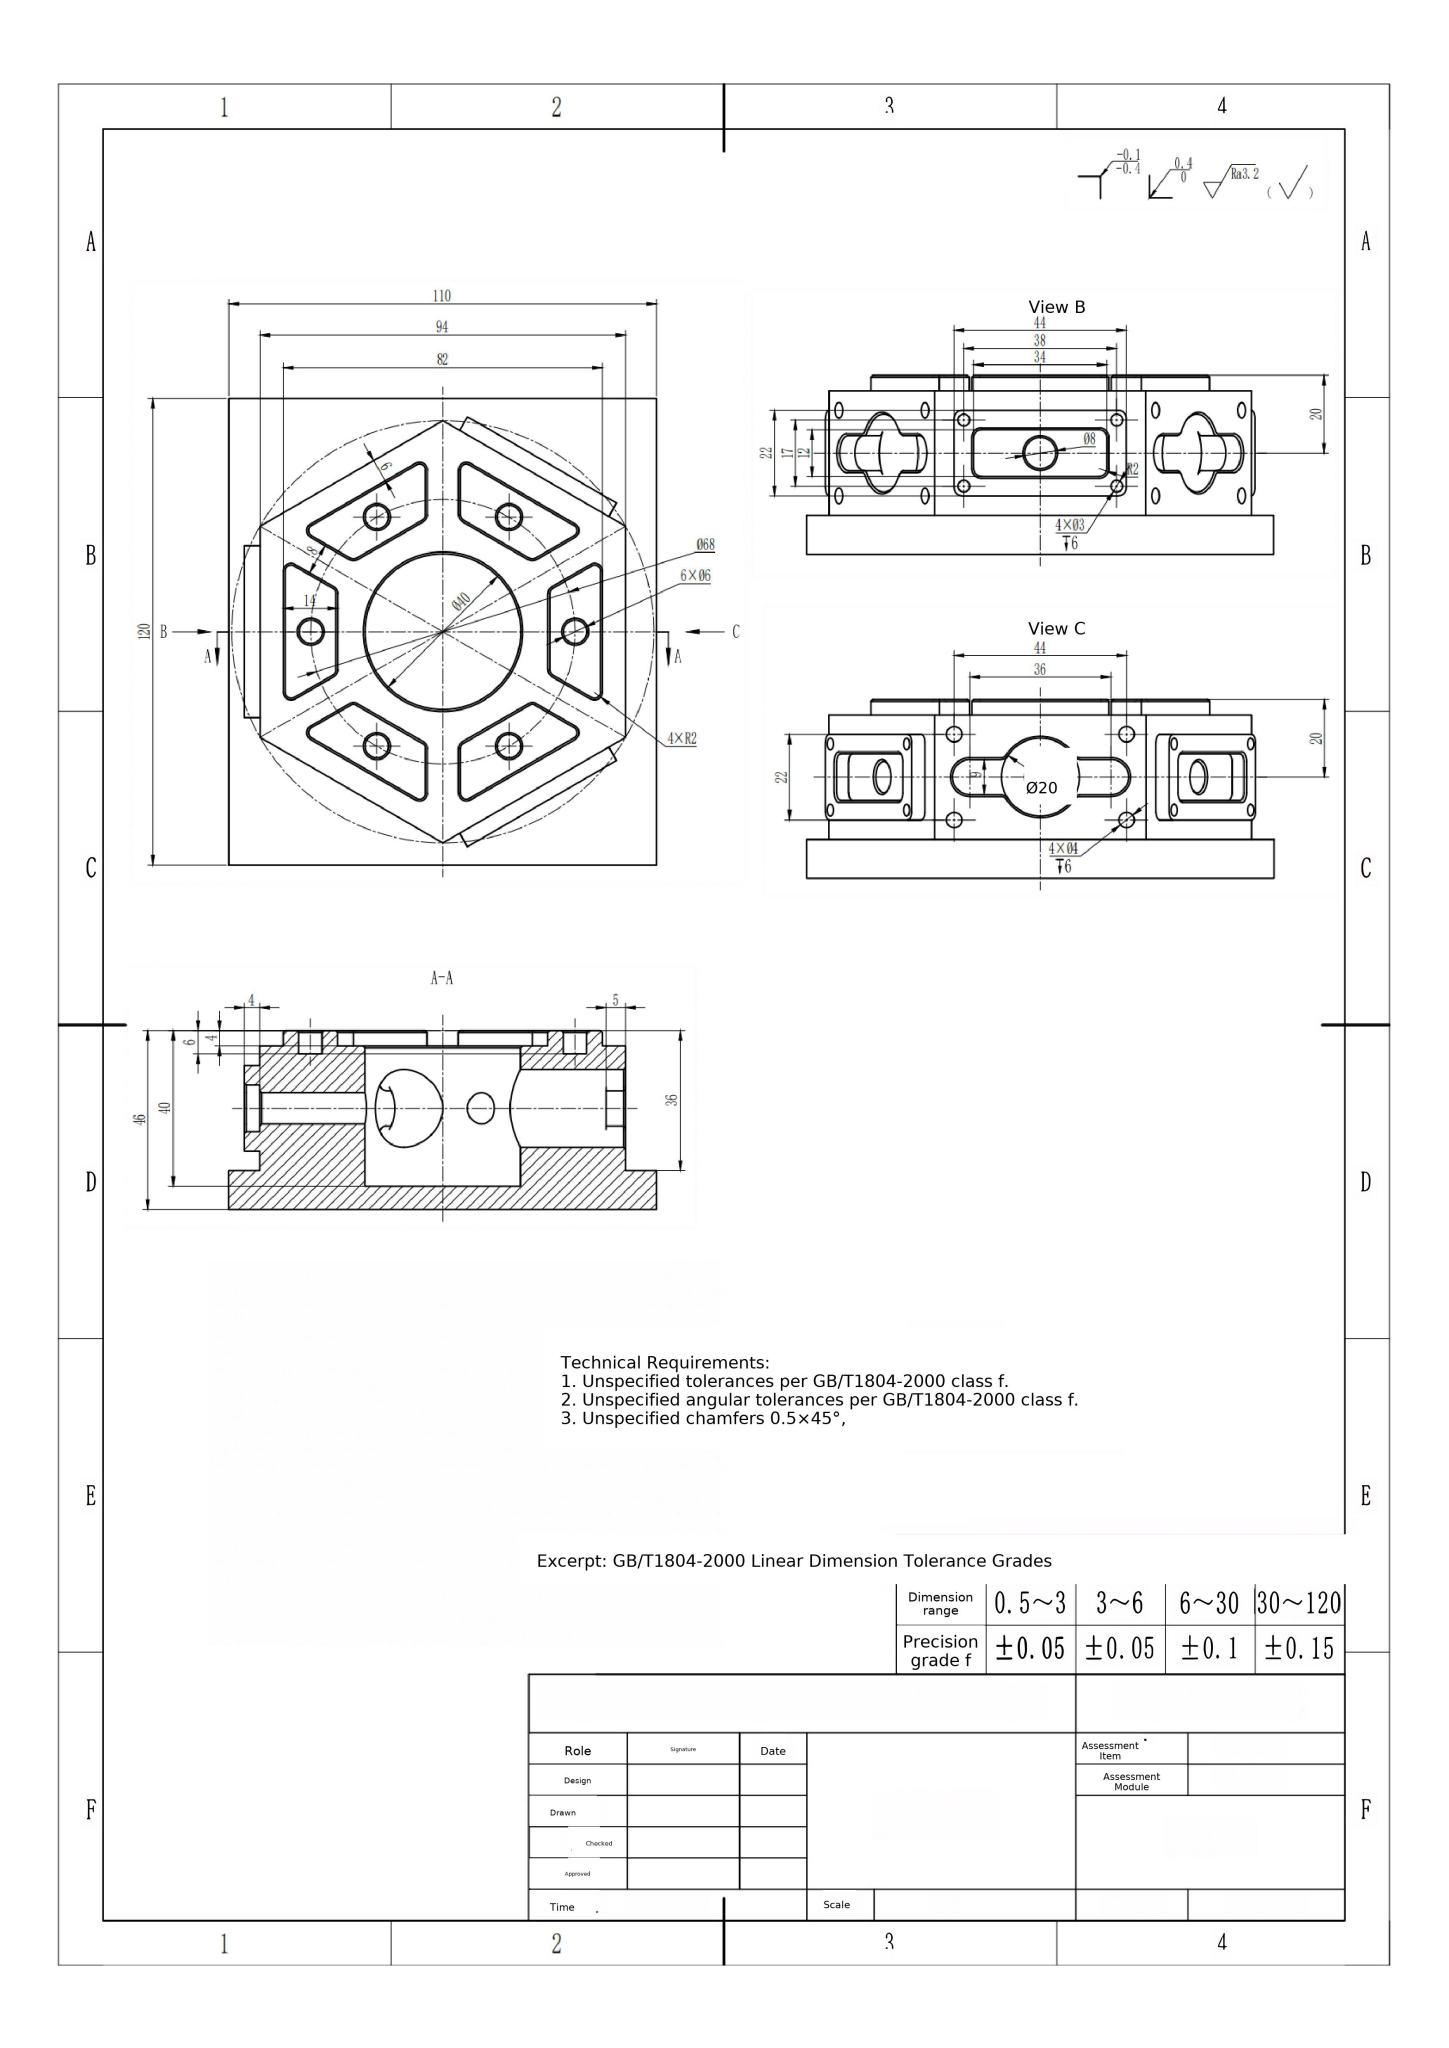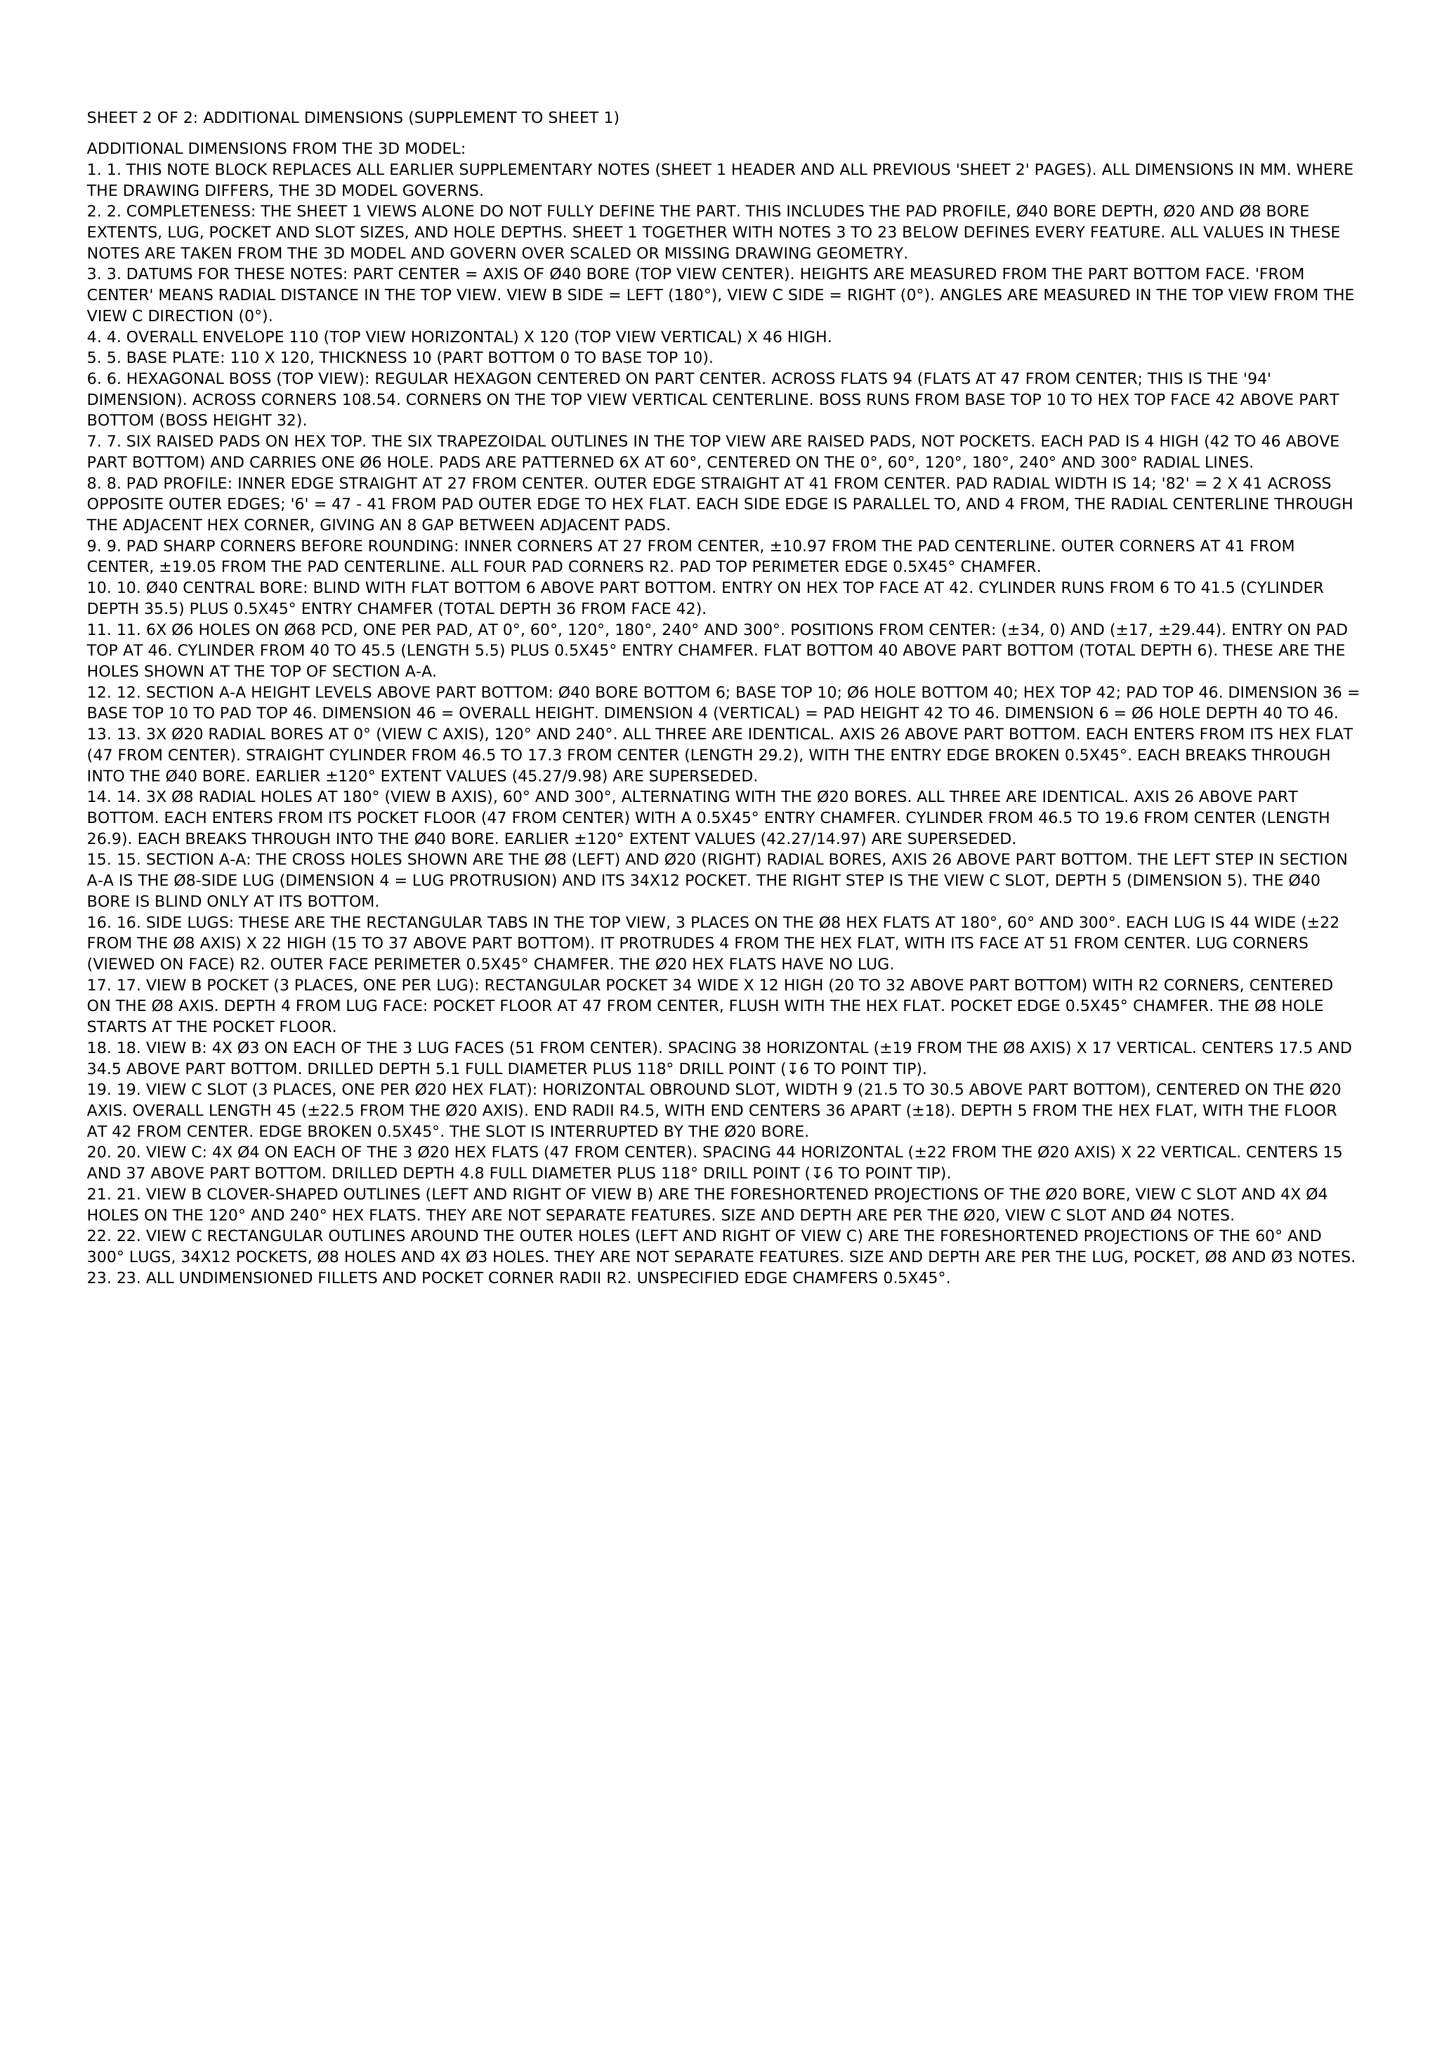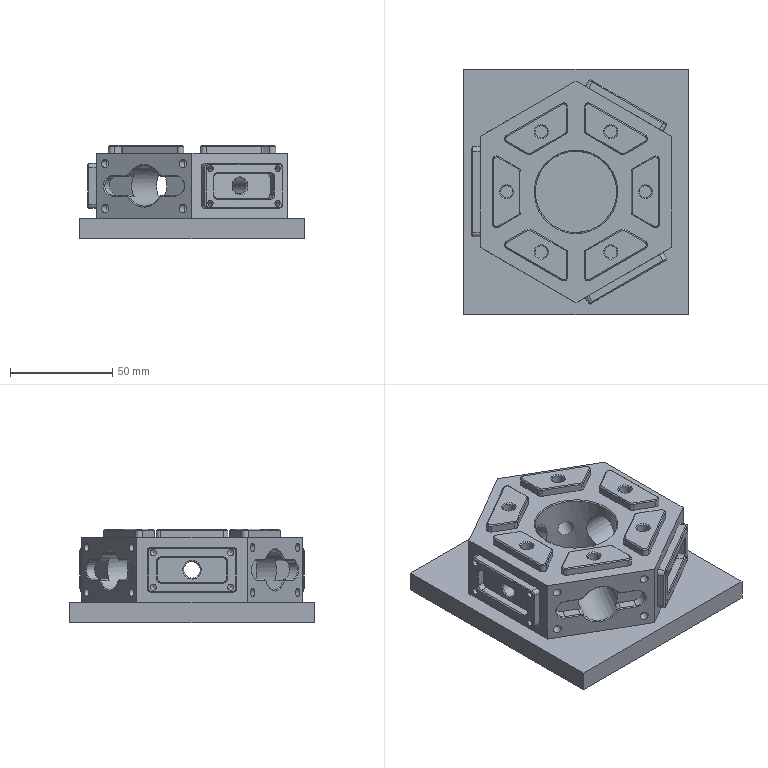Part | NX | mm | 1 solid | 367 faces | box 110 x 120 x 46 mm | volume 312439 mm3 | plane 158 | cone 106 | cylinder 103 | commonest cylinder face diameters 4 x72 3 x12 6 x6 9 x6 8 x3 20 x3 40 x1